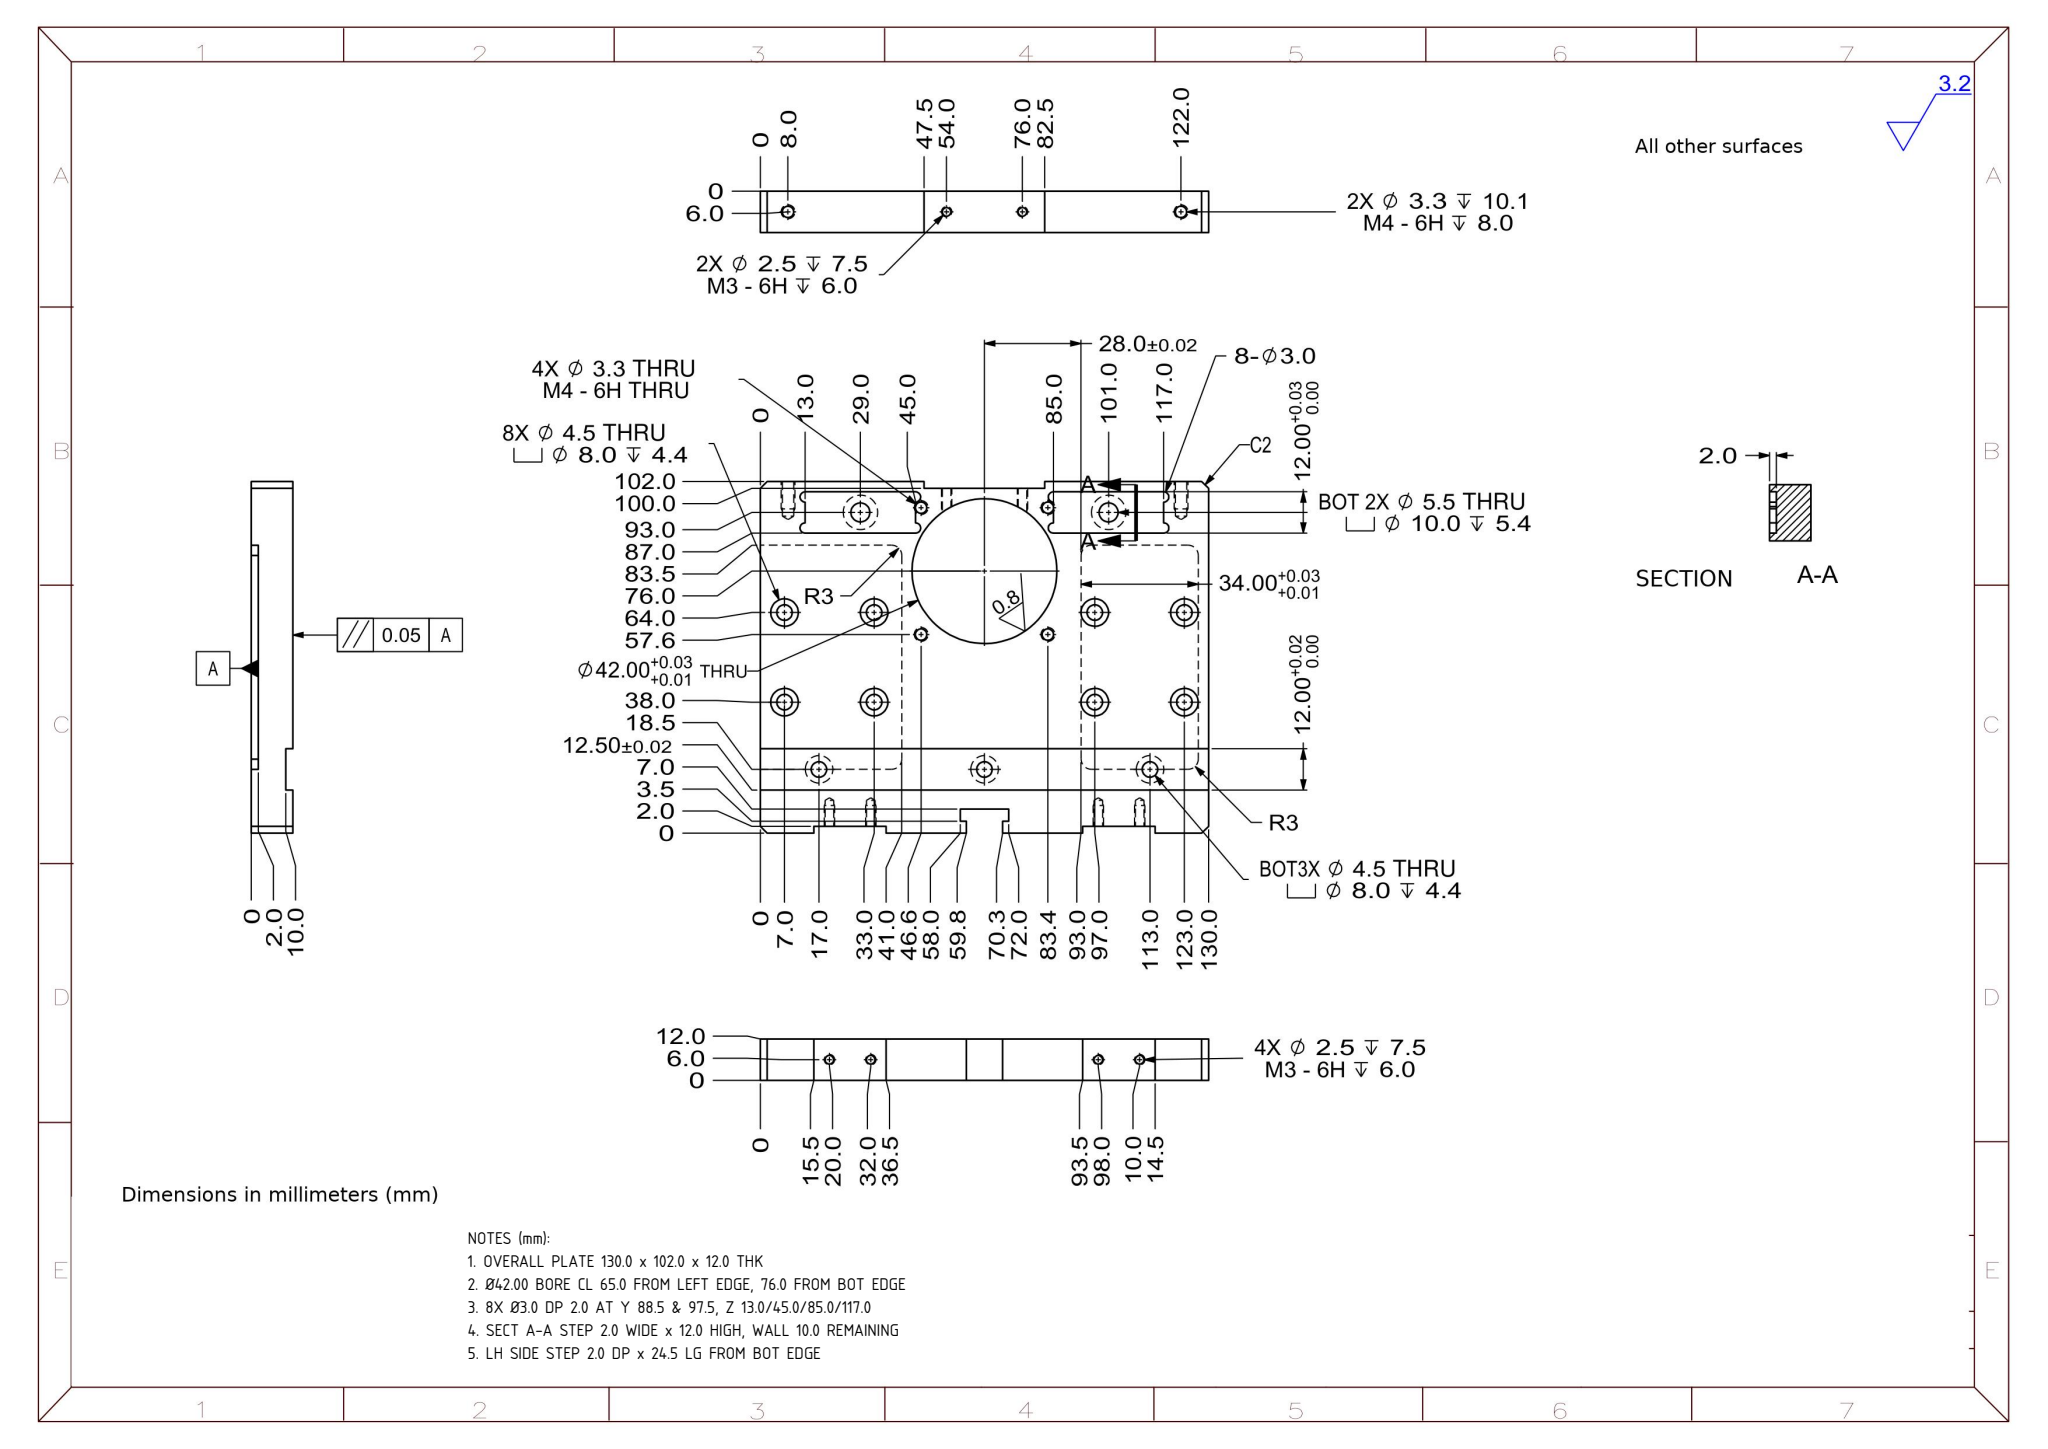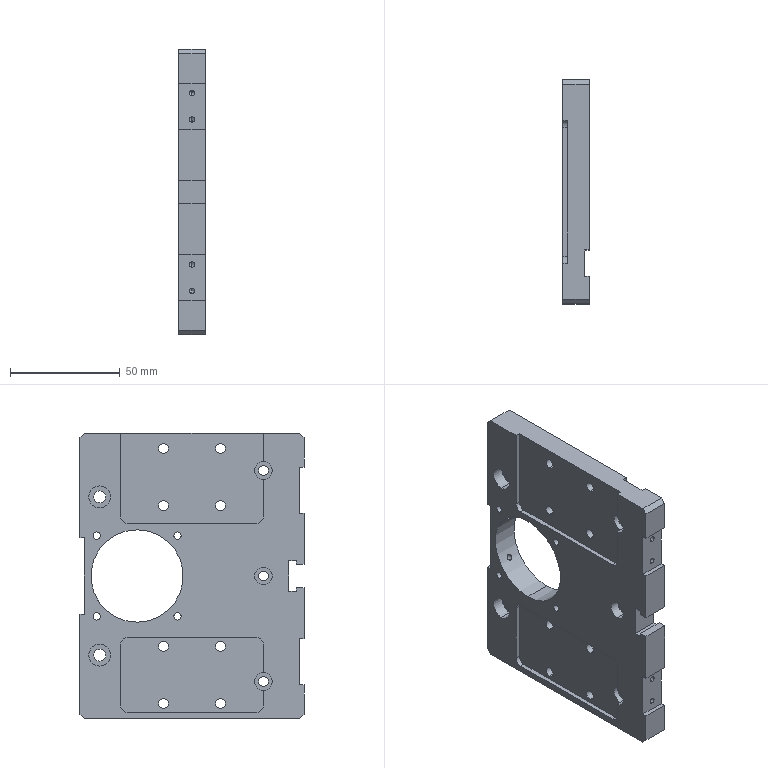Part | SolidWorks | mm | 1 solid | 178 faces | box 12 x 102 x 130 mm | volume 119902 mm3 | cylinder 96 | plane 70 | cone 12 | commonest cylinder face diameters 8 x22 4.5 x22 3.3 x12 2.5 x12 3 x12 6 x6 10 x4 5.5 x4
Drawing notes:
OVERALL PLATE 130.0 x 102.0 x 12.0 THK | from the solid: bbox 130 x 102; bore len 12.0 THRU
Ø42.00 BORE CL 65.0 FROM LEFT EDGE, 76.0 FROM BOT EDGE | from the solid: Cyl dia 42.0 axis x at (y=76.0, z=65.0), length 12.0 THRU; bbox 130 x 102
8X Ø3.0 DP 2.0 AT Y 88.5 & 97.5, Z 13.0/45.0/85.0/117.0 | from the solid: Eight 3.0 dia cyls, axis x, len 2.0, at y=88.5/97.5 and z=13,45,85,117
SECT A-A STEP 2.0 WIDE x 12.0 HIGH, WALL 10.0 REMAINING | from the solid: y planes 87.0 & 99.0 (12.0 apart); x planes 10.0 and 12.0 give 2.0 step
LH SIDE STEP 2.0 DP x 24.5 LG FROM BOT EDGE | from the solid: Single y plane at 24.5 ends step; x planes 10.0/12.0 = 2.0 deep recess
build123d program:
from build123d import *

# Parameters (mm, degrees)
SKETCH1_W                                       = 130
SKETCH1_H                                       = 102
BOSS_EXTRUDE1_DEPTH                             = 6
CHAMFER1_SIZE                                   = 2
CUT_EXTRUDE1_DEPTH                              = 34
SKETCH3_R                                       = 21
CUT_EXTRUDE2_DEPTH                              = 84.487
SKETCH4_W                                       = 130
SKETCH4_H                                       = 12
CUT_EXTRUDE3_DEPTH                              = 2
SKETCH5_W                                       = 32
SKETCH5_H                                       = 12
CUT_EXTRUDE4_DEPTH                              = 2
SKETCH6_W                                       = 12
SKETCH6_H                                       = 35
CUT_EXTRUDE5_DEPTH                              = 2
SKETCH7_W                                       = 12
SKETCH7_H                                       = 21
CUT_EXTRUDE6_DEPTH                              = 2
SKETCH8_R                                       = 1.5
CUT_EXTRUDE7_DEPTH                              = 2
CUT_EXTRUDE8_DEPTH                              = 2
M4_HEX_SOCKET_HEAD_CAP_SCREW_CBORE1_D           = 4.5
M4_HEX_SOCKET_HEAD_CAP_SCREW_CBORE1_CBORE_D     = 8
M4_HEX_SOCKET_HEAD_CAP_SCREW_CBORE1_CBORE_DEPTH = 4.4
M5_HEX_SOCKET_HEAD_CAP_SCREW_CBORE1_D           = 5.5
M5_HEX_SOCKET_HEAD_CAP_SCREW_CBORE1_CBORE_D     = 10
M5_HEX_SOCKET_HEAD_CAP_SCREW_CBORE1_CBORE_DEPTH = 5.4
M3_TAPPED_HOLE1_D                               = 2.5
M3_TAPPED_HOLE1_DEPTH                           = 7.5
M3_TAPPED_HOLE1_TIP                             = 0.7511
M3_TAPPED_HOLE2_D                               = 2.5
M3_TAPPED_HOLE2_DEPTH                           = 7.5
M3_TAPPED_HOLE2_TIP                             = 0.7511
M4_TAPPED_HOLE1_D                               = 3.3
M4_HEX_SOCKET_HEAD_CAP_SCREW_CBORE2_D           = 4.5
M4_HEX_SOCKET_HEAD_CAP_SCREW_CBORE2_CBORE_D     = 8
M4_HEX_SOCKET_HEAD_CAP_SCREW_CBORE2_CBORE_DEPTH = 4.4
M4_TAPPED_HOLE2_D                               = 3.3
M4_TAPPED_HOLE2_DEPTH                           = 10.1
M4_TAPPED_HOLE2_TIP                             = 0.9914


with BuildPart() as part:
    # Sketch1 → Boss-Extrude1 (new, symmetric)
    with BuildSketch(Plane(origin=(0, 0, 0), x_dir=(0, 0, -1), z_dir=(1, 0, 0))):
        Rectangle(SKETCH1_W, SKETCH1_H)
    extrude(amount=BOSS_EXTRUDE1_DEPTH, both=True)

    # Chamfer1
    chamfer1_edges = [part.edges().sort_by_distance(p)[0] for p in [
        (0, 51, 65),
        (0, 51, -65),
        (0, -51, -65),
        (0, -51, 65),
    ]]
    chamfer(chamfer1_edges, length=CHAMFER1_SIZE)

    # Sketch2 → Cut-Extrude1 (cut)
    with BuildSketch(Plane(origin=(6, 0, 0), x_dir=(0, 0, -1), z_dir=(1, 0, 0))):
        Polygon((7, -44), (-7, -44), (-7, -47.5), (-5.25, -47.5), (-5.25, -51), (5.25, -51), (5.25, -47.5), (7, -47.5), align=None)
    extrude(amount=-CUT_EXTRUDE1_DEPTH, mode=Mode.SUBTRACT)

    # Sketch3 → Cut-Extrude2 (cut, through all)
    with BuildSketch(Plane(origin=(6, 0, 0), x_dir=(0, 0, -1), z_dir=(1, 0, 0))):
        with Locations((0, 25)):
            Circle(SKETCH3_R)
    extrude(amount=-CUT_EXTRUDE2_DEPTH, mode=Mode.SUBTRACT)

    # Sketch4 → Cut-Extrude3 (cut)
    with BuildSketch(Plane(origin=(6, 0, 0), x_dir=(0, 0, -1), z_dir=(1, 0, 0))):
        with Locations((0, -32.5)):
            Rectangle(SKETCH4_W, SKETCH4_H)
    extrude(amount=-CUT_EXTRUDE3_DEPTH, mode=Mode.SUBTRACT)

    # Sketch5 → Cut-Extrude4 (cut)
    with BuildSketch(Plane(origin=(6, 0, 0), x_dir=(0, 0, -1), z_dir=(1, 0, 0))):
        with Locations((36, 42)):
            Rectangle(SKETCH5_W, SKETCH5_H)
        with Locations((-36, 42)):
            Rectangle(SKETCH5_W, SKETCH5_H)
    extrude(amount=-CUT_EXTRUDE4_DEPTH, mode=Mode.SUBTRACT)

    # Sketch6 → Cut-Extrude5 (cut)
    with BuildSketch(Plane(origin=(0, 51, 0), x_dir=(1, 0, 0), z_dir=(0, 1, 0))):
        Rectangle(SKETCH6_W, SKETCH6_H)
    extrude(amount=-CUT_EXTRUDE5_DEPTH, mode=Mode.SUBTRACT)

    # Sketch7 → Cut-Extrude6 (cut)
    with BuildSketch(Plane(origin=(0, -51, 0), x_dir=(-1, 0, 0), z_dir=(0, -1, 0))):
        with Locations((0, -39)):
            Rectangle(SKETCH7_W, SKETCH7_H)
        with Locations((0, 39)):
            Rectangle(SKETCH7_W, SKETCH7_H)
    extrude(amount=-CUT_EXTRUDE6_DEPTH, mode=Mode.SUBTRACT)

    # Sketch8 → Cut-Extrude7 (cut)
    with BuildSketch(Plane(origin=(6, 0, 0), x_dir=(0, 0, -1), z_dir=(1, 0, 0))):
        with Locations((-52, 46.5)):
            Circle(SKETCH8_R)
        with Locations((-52, 37.5)):
            Circle(SKETCH8_R)
        with Locations((-20, 46.5)):
            Circle(SKETCH8_R)
        with Locations((-20, 37.5)):
            Circle(SKETCH8_R)
        with Locations((20, 46.5)):
            Circle(SKETCH8_R)
        with Locations((20, 37.5)):
            Circle(SKETCH8_R)
        with Locations((52, 46.5)):
            Circle(SKETCH8_R)
        with Locations((52, 37.5)):
            Circle(SKETCH8_R)
    extrude(amount=-CUT_EXTRUDE7_DEPTH, mode=Mode.SUBTRACT)

    # Sketch9 → Cut-Extrude8 (cut)
    with BuildSketch(Plane.ZY.offset(6)):
        with BuildLine():
            Line((-59, 32.5), (-31, 32.5))
            ThreePointArc((-31, 32.5), (-28.879, 31.621), (-28, 29.5))
            Line((-28, 29.5), (-28, -29.5))
            ThreePointArc((-28, -29.5), (-28.879, -31.621), (-31, -32.5))
            Line((-31, -32.5), (-59, -32.5))
            ThreePointArc((-59, -32.5), (-61.121, -31.621), (-62, -29.5))
            Line((-62, -29.5), (-62, 29.5))
            ThreePointArc((-62, 29.5), (-61.121, 31.621), (-59, 32.5))
        make_face()
        with BuildLine():
            Line((27, 32.5), (65, 32.5))
            Line((65, 32.5), (65, -32.5))
            Line((65, -32.5), (27, -32.5))
            ThreePointArc((27, -32.5), (24.879, -31.621), (24, -29.5))
            Line((24, -29.5), (24, 29.5))
            ThreePointArc((24, 29.5), (24.879, 31.621), (27, 32.5))
        make_face()
    extrude(amount=-CUT_EXTRUDE8_DEPTH, mode=Mode.SUBTRACT)

    # M4 Hex Socket Head Cap Screw CBORE1 (through all)
    with Locations(Plane(origin=(6, 0, 0), x_dir=(0, 0, -1), z_dir=(1, 0, 0))):
        with Locations((-58, 13), (-32, 13), (-58, -13), (-32, -13), (32, 13), (58, 13), (32, -13), (58, -13)):
            CounterBoreHole(M4_HEX_SOCKET_HEAD_CAP_SCREW_CBORE1_D / 2, M4_HEX_SOCKET_HEAD_CAP_SCREW_CBORE1_CBORE_D / 2, M4_HEX_SOCKET_HEAD_CAP_SCREW_CBORE1_CBORE_DEPTH)

    # M5 Hex Socket Head Cap Screw CBORE1 (through all)
    with Locations(Plane.ZY.offset(6)):
        with Locations((-36, 42), (36, 42)):
            CounterBoreHole(M5_HEX_SOCKET_HEAD_CAP_SCREW_CBORE1_D / 2, M5_HEX_SOCKET_HEAD_CAP_SCREW_CBORE1_CBORE_D / 2, M5_HEX_SOCKET_HEAD_CAP_SCREW_CBORE1_CBORE_DEPTH)

    # M3 Tapped Hole1
    with Locations(Plane(origin=(0, -49, 0), x_dir=(-1, 0, 0), z_dir=(0, -1, 0))):
        with Locations((0, -45), (0, -33), (0, 33), (0, 45)):
            Hole(M3_TAPPED_HOLE1_D / 2, depth=M3_TAPPED_HOLE1_DEPTH)
            with Locations((0, 0, -(M3_TAPPED_HOLE1_DEPTH + M3_TAPPED_HOLE1_TIP / 2))):  # 118° drill point
                Cone(0, M3_TAPPED_HOLE1_D / 2, M3_TAPPED_HOLE1_TIP, mode=Mode.SUBTRACT)

    # M3 Tapped Hole2
    with Locations(Plane(origin=(0, 49, 0), x_dir=(1, 0, 0), z_dir=(0, 1, 0))):
        with Locations((0, -11), (0, 11)):
            Hole(M3_TAPPED_HOLE2_D / 2, depth=M3_TAPPED_HOLE2_DEPTH)
            with Locations((0, 0, -(M3_TAPPED_HOLE2_DEPTH + M3_TAPPED_HOLE2_TIP / 2))):  # 118° drill point
                Cone(0, M3_TAPPED_HOLE2_D / 2, M3_TAPPED_HOLE2_TIP, mode=Mode.SUBTRACT)

    # M4 Tapped Hole1 (through all)
    with Locations(Plane.ZY.offset(6)):
        with Locations((-18.385, 43.385), (-18.385, 6.615), (18.385, 6.615), (18.385, 43.385)):
            Hole(M4_TAPPED_HOLE1_D / 2)

    # M4 Hex Socket Head Cap Screw CBORE2 (through all)
    with Locations(Plane.ZY.offset(6)):
        with Locations((0, -32.5), (48, -32.5), (-48, -32.5)):
            CounterBoreHole(M4_HEX_SOCKET_HEAD_CAP_SCREW_CBORE2_D / 2, M4_HEX_SOCKET_HEAD_CAP_SCREW_CBORE2_CBORE_D / 2, M4_HEX_SOCKET_HEAD_CAP_SCREW_CBORE2_CBORE_DEPTH)

    # M4 Tapped Hole2
    with Locations(Plane(origin=(0, 51, 0), x_dir=(1, 0, 0), z_dir=(0, 1, 0))):
        with Locations((0, -57), (0, 57)):
            Hole(M4_TAPPED_HOLE2_D / 2, depth=M4_TAPPED_HOLE2_DEPTH)
            with Locations((0, 0, -(M4_TAPPED_HOLE2_DEPTH + M4_TAPPED_HOLE2_TIP / 2))):  # 118° drill point
                Cone(0, M4_TAPPED_HOLE2_D / 2, M4_TAPPED_HOLE2_TIP, mode=Mode.SUBTRACT)


solid = part.part